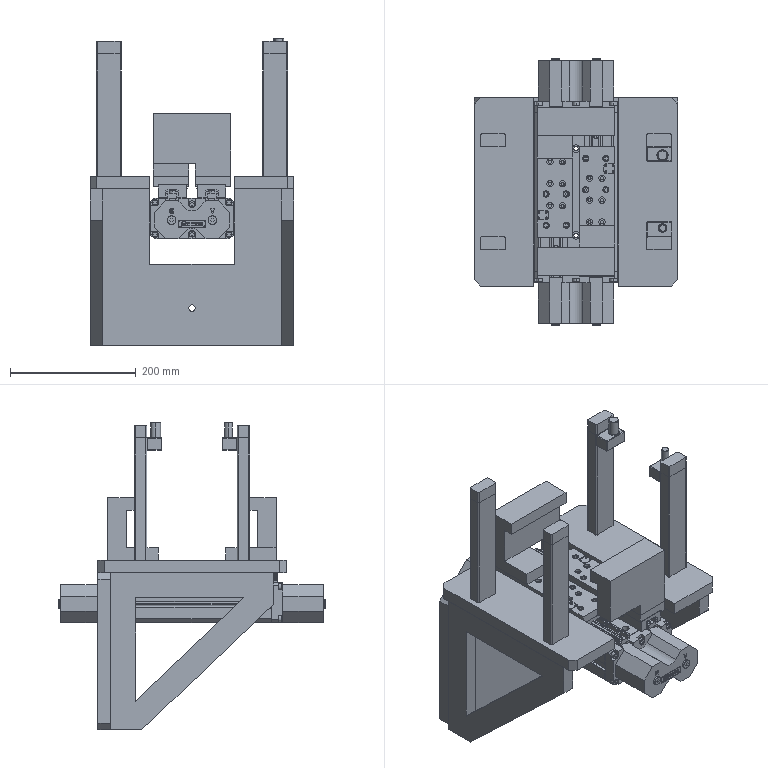Assembly | SolidWorks | mm | 25 component files | 26 solids | 4041 faces | box 325 x 424.4 x 490 mm | volume 8958656 mm3 | plane 3240 | cylinder 593 | cone 112 | spline 96 | commonest cylinder face diameters 10 x100 4 x54 4.917 x48 0.4 x48 4.134 x44 9.48 x38 5 x34 3.2 x32
Bill of materials:
AngleSupport | 2 | Aviation Aluminum-7075 | Flat triangular frame: a right-triangle outline plate of uniform thickness with a matching triangular through-opening, leaving three straight members of roughly equal width.
LocatingPinA | 1 | Aviation Aluminum-7075 | Rectangular block with chamfered edges and one cylindrical pin standing up from its top face, placed off-center. The pin has a chamfered tip and a small chamfer or fillet ring where it meets the block.
LocatingPinB | 1 | Aviation Aluminum-7075 | Rectangular block with chamfered edges and one off-center cylindrical pin with a chamfered tip and a ring at its base. Similar to unnamed part, but the pin is visibly smaller in diameter.
ParallelGripperFingerA | 2 | Aviation Aluminum-7075 | Stepped prismatic block made of offset rectangular sections: a tall main slab, a lower ledge projecting to one side, and a small overhanging lip at the top. The side and front profiles are L- or Z-shaped.
Pillar | 4 | Aviation Aluminum-7075 | Long rectangular bar or post with small rounded longitudinal edges. Its cross-section is a rounded rectangle.
RobotGripperBasePlateAA | 1 | Aviation Aluminum-7075 | Two separate thin rectangular plates arranged side by side in one model. Each has chamfered corners on one end and two shallow L-shaped grooves or marks engraved in the top face.
RobotGripperBasePlateB | 1 | Aviation Aluminum-7075 | Flat plate with chamfered corners, one wide rectangular U-notch cut in from one edge, and one small round through-hole in the solid section below the notch.
SCHUNK-1005128 Gehaeuse PHL-50-060-S,0 | 1 |  | Elongated multi-feature body, likely a composite of several shapes. Two parallel faceted (octagonal-section) bars with concave grooves run the full length. A central raised rectangular deck covers part of the length; it has a row of small holes, several larger holes, and longitudinal slots. End blocks carry small round heads. The opposite face shows a plate with circular bosses and notches on one edge.
SCHUNK-5521418 Abdeckblech PHL-50-060 | 2 |  | Long thin flat strip with rounded ends. A raised rounded-end pad sits at mid-length, with a rectangular through-slot and two small cylindrical bosses that have small central recesses.
SCHUNK-5521421 Gleitschiene PHL-G-50-060 | 2 |  | Long straight rail-like profile with a constant cross-section. Each flank has a serrated (multi-tooth V-groove) edge, there is a central recess on top and wide feet with a central channel underneath, and a row of evenly spaced counterbored holes runs along its length.
SCHUNK-55xxxxx Grundbacke PHL-G 50 | 2 |  | Elongated block with a T-shaped cross-section. A wide top plate sits over a narrower body containing an internal channel with serrated V-tooth walls. The top has many counterbored holes, some showing socket-shaped recesses, plus small holes and two transverse grooves. Small round holes are on the side faces, and a central lower section projects below.
SCHUNK-9905503 Typenschild 11x43x0.3 | 2 |  | Very thin flat stadium-shaped (obround) plate or shim with fully rounded ends and no internal features.
WearBlock | 4 | H62 | Solid rectangular block with rounded vertical edges; it looks like a rounded-rectangle profile extruded straight with flat top and bottom faces. The plan view is about 2:1, and the height looks roughly equal to the short side.
Mates:
1. coincident | RobotGripperBasePlateAA-1 face at (-161.87, -408.626, 492.215) dir (0, 0, 1) | Pillar-1 face at (-197.87, -408.626, 492.215) dir (0, 0, -1)
2. coincident | RobotGripperBasePlateAA-1 face at (-161.87, -406.626, 492.215) dir (0, -1, 0) | Pillar-1 face at (-161.87, -406.626, 492.215) dir (0, 1, 0)
3. coincident | RobotGripperBasePlateAA-1 face at (-199.87, -408.626, 492.215) dir (1, 0, 0) | Pillar-1 face at (-199.87, -408.626, 492.215) dir (-1, 0, 0)
4. coincident | Pillar-1 face at (-197.87, -408.626, 692.215) dir (0, 0, 1) | WearBlock-1 face at (-161.87, -424.626, 692.215) dir (0, 0, -1)
5. coincident | Pillar-1 face at (-161.87, -426.626, 492.215) dir (0, -1, 0) | WearBlock-1 face at (-197.87, -426.626, 692.215) dir (0, -1, 0)
6. coincident | Pillar-1 face at (-199.87, -408.626, 492.215) dir (-1, 0, 0) | WearBlock-1 face at (-199.87, -424.626, 692.215) dir (-1, 0, 0)
7. coincident | RobotGripperBasePlateAA-1 face at (-47.37, -334.626, 477.215) dir (0, 0, -1) | RobotGripperBasePlateB-1 face at (-209.87, -204.626, 477.215) dir (0, 0, 1)
8. coincident | RobotGripperBasePlateAA-1 face at (115.13, -184.626, 497.215) dir (0, 1, 0) | RobotGripperBasePlateB-1 face at (-47.37, -184.626, 352.215) dir (0, 1, 0)
9. coincident | RobotGripperBasePlateAA-1 face at (115.13, -484.626, 497.215) dir (1, 0, 0) | RobotGripperBasePlateB-1 face at (115.13, -204.626, 477.215) dir (1, 0, 0)
10. coincident | RobotGripperBasePlateB-1 face at (-47.37, -204.626, 352.215) dir (0, -1, 0) | AngleSupport-1 face at (95.13, -204.626, 477.215) dir (0, 1, 0)
11. coincident | RobotGripperBasePlateAA-1 face at (-47.37, -334.626, 477.215) dir (0, 0, -1) | AngleSupport-1 face at (95.13, -464.626, 477.215) dir (0, 0, 1)
12. coincident | RobotGripperBasePlateAA-1 face at (115.13, -484.626, 497.215) dir (1, 0, 0) | AngleSupport-1 face at (115.13, -204.626, 227.215) dir (1, 0, 0)
13. coincident | RobotGripperBasePlateAA-1 face at (-47.37, -334.626, 477.215) dir (0, 0, -1) | AngleSupport-2 face at (-209.87, -464.626, 477.215) dir (0, 0, 1)
14. coincident | RobotGripperBasePlateB-1 face at (-47.37, -204.626, 352.215) dir (0, -1, 0) | AngleSupport-2 face at (-209.87, -204.626, 477.215) dir (0, 1, 0)
15. coincident | RobotGripperBasePlateAA-1 face at (-209.87, -484.626, 497.215) dir (-1, 0, 0) | AngleSupport-2 face at (-209.87, -204.626, 227.215) dir (-1, 0, 0)
16. width | RobotGripperBasePlateAA-1 face at (-209.87, -484.626, 497.215) dir (-1, 0, 0) | RobotGripperBasePlateAA-1 face at (115.13, -484.626, 497.215) dir (1, 0, 0) | SCHUNK-0308183PHL-G50-060-S,00000000LinearGripper-1/SCHUNK-1005128 Gehaeuse PHL-50-060-S,0-1 face at (18.63, -208.426, 456.415) dir (1, 0, 0) | SCHUNK-0308183PHL-G50-060-S,00000000LinearGripper-1/SCHUNK-1005128 Gehaeuse PHL-50-060-S,0-1 face at (-113.37, -208.426, 403.915) dir (-1, 0, 0)
17. width | RobotGripperBasePlateAA-1 face at (115.13, -484.626, 497.215) dir (0, -1, 0) | RobotGripperBasePlateAA-1 face at (115.13, -184.626, 497.215) dir (0, 1, 0) | SCHUNK-0308183PHL-G50-060-S,00000000LinearGripper-1/SCHUNK-1005128 Gehaeuse PHL-50-060-S,0-1 face at (-47.37, -125.426, 397.415) dir (0, 1, 0) | SCHUNK-0308183PHL-G50-060-S,00000000LinearGripper-1/SCHUNK-1005128 Gehaeuse PHL-50-060-S,0-1 face at (-47.37, -543.826, 397.415) dir (0, -1, 0)
18. coincident | RobotGripperBasePlateAA-1 face at (-47.37, -334.626, 497.215) dir (0, 0, 1) | SCHUNK-0308183PHL-G50-060-S,00000000LinearGripper-1/SCHUNK-55xxxxx Grundbacke PHL-G 50-2 face at (-41.87, -261.626, 497.215) dir (0, 0, 1)
19. coincident | SCHUNK-0308183PHL-G50-060-S,00000000LinearGripper-1/SCHUNK-55xxxxx Grundbacke PHL-G 50-1 face at (-52.87, -407.626, 497.215) dir (0, 0, 1) | ParallelGripperFingerA-1 face at (-80.87, -240.626, 497.215) dir (0, 0, -1)
20. coincident | SCHUNK-0308183PHL-G50-060-S,00000000LinearGripper-1/SCHUNK-55xxxxx Grundbacke PHL-G 50-1 face at (-78.87, -200.626, 463.115) dir (0, 1, 0) | ParallelGripperFingerA-1 face at (-52.87, -200.626, 517.215) dir (0, 1, 0)
21. coincident | SCHUNK-0308183PHL-G50-060-S,00000000LinearGripper-1/SCHUNK-55xxxxx Grundbacke PHL-G 50-1 face at (-108.87, -407.626, 497.215) dir (-1, 0, 0) | ParallelGripperFingerA-1 face at (-108.87, -200.626, 517.215) dir (-1, 0, 0)
22. coincident | SCHUNK-0308183PHL-G50-060-S,00000000LinearGripper-1/SCHUNK-55xxxxx Grundbacke PHL-G 50-2 face at (-41.87, -261.626, 497.215) dir (0, 0, 1) | ParallelGripperFingerA-2 face at (-13.87, -428.626, 497.215) dir (0, 0, -1)
23. coincident | SCHUNK-0308183PHL-G50-060-S,00000000LinearGripper-1/SCHUNK-55xxxxx Grundbacke PHL-G 50-2 face at (-15.87, -468.626, 463.115) dir (0, -1, 0) | ParallelGripperFingerA-2 face at (-41.87, -468.626, 517.215) dir (0, -1, 0)
24. coincident | SCHUNK-0308183PHL-G50-060-S,00000000LinearGripper-1/SCHUNK-55xxxxx Grundbacke PHL-G 50-2 face at (14.13, -261.626, 497.215) dir (1, 0, 0) | ParallelGripperFingerA-2 face at (14.13, -468.626, 517.215) dir (1, 0, 0)
25. coincident | Pillar-4 face at (103.13, -262.626, 492.215) dir (0, -1, 0) | LocatingPinA-1 face at (85.13, -262.626, 682.215) dir (0, 1, 0)
26. coincident | Pillar-4 edge at (103.13, -262.626, 692.215) dir (-1, 0, 0) | LocatingPinA-1 face at (65.13, -286.626, 692.215) dir (0, 0, 1)
27. coincident | Pillar-4 face at (105.13, -244.626, 492.215) dir (1, 0, 0) | LocatingPinA-1 face at (105.13, -286.626, 692.215) dir (1, 0, 0)
28. coincident | Pillar-3 face at (103.13, -406.626, 492.215) dir (0, 1, 0) | LocatingPinB-1 face at (85.13, -406.626, 682.215) dir (0, -1, 0)
29. coincident | Pillar-3 face at (105.13, -408.626, 492.215) dir (1, 0, 0) | LocatingPinB-1 face at (105.13, -382.626, 692.215) dir (1, 0, 0)
30. coincident | Pillar-3 edge at (67.13, -406.626, 692.215) dir (1, 0, 0) | LocatingPinB-1 face at (105.13, -382.626, 692.215) dir (0, 0, 1)